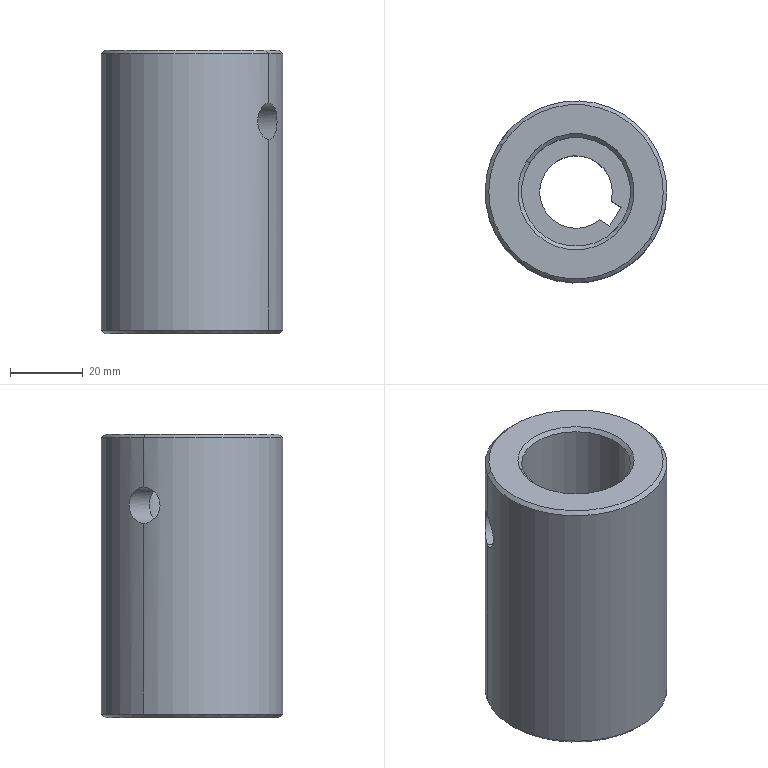Component | SolidWorks | 24-1 | 1 solid | 24 faces | box 50 x 50 x 78 mm | volume 107825 mm3 | cylinder 10 | cone 8 | plane 6 | commonest cylinder face diameters 10 x4 30 x2 20 x2 50 x2
build123d program:
from build123d import *

# Parameters (mm, degrees)
SKETCH1_R            = 25
BOSS_EXTRUDE1_DEPTH  = 78
CUT_EXTRUDE1_DEPTH   = 31
SKETCH3_R            = 15
CUT_EXTRUDE2_DEPTH   = 47
CUT_SWEEP1_PROFILE_R = 5
CHAMFER1_SIZE        = 1
CHAMFER2_SIZE        = 1
CHAMFER3_SIZE        = 1


with BuildPart() as part:
    # Sketch1 → Boss-Extrude1 (new body)
    with BuildSketch(Plane(origin=(0, 0, 0), x_dir=(1, 0, 0), z_dir=(0, 1, 0))):
        with Locations(Location((0, 0, 0), (0, 0, 270))):
            Circle(SKETCH1_R)
    extrude(amount=BOSS_EXTRUDE1_DEPTH)

    # Sketch2 → Cut-Extrude1 (cut)
    with BuildSketch(Plane(origin=(0, 78, 0), x_dir=(1, 0, 0), z_dir=(0, 1, 0))):
        with BuildLine():
            Line((3, 12.8), (-3, 12.8))
            Line((-3, 12.8), (-3, 9.539))
            ThreePointArc((-3, 9.539), (0, -10), (3, 9.539))
            Line((3, 9.539), (3, 12.8))
        make_face()
    extrude(amount=-CUT_EXTRUDE1_DEPTH, mode=Mode.SUBTRACT)

    # Sketch3 → Cut-Extrude2 (cut)
    with BuildSketch(Plane(origin=(0, 47, 0), x_dir=(1, 0, 0), z_dir=(0, 1, 0))):
        with Locations(Location((0, 0, 0), (0, 0, 270))):
            Circle(SKETCH3_R)
    extrude(amount=-CUT_EXTRUDE2_DEPTH, mode=Mode.SUBTRACT)

    # Cut-Sweep1: sweep along a path in Sketch4
    with BuildLine(Plane(origin=(0, 0, 0), x_dir=(0, 0, -1), z_dir=(1, 0, 0))) as cut_sweep1_path:
        Line((45.424, 19.5), (-33.131, 19.5))
    # Cut-Sweep1 profile (on start of the path) → Cut-Sweep1 (sweep, cut)
    with BuildSketch(Plane(origin=(0, 19.5, -45.424), x_dir=(0, 1, 0), z_dir=(0, 0, 1))):
        Circle(CUT_SWEEP1_PROFILE_R)
    sweep(path=cut_sweep1_path.line, mode=Mode.SUBTRACT)

    # Chamfer1
    chamfer1_edges = [part.edges().sort_by_distance(p)[0] for p in [
        (0, 0, -25),
        (0, 78, -25),
    ]]
    chamfer(chamfer1_edges, length=CHAMFER1_SIZE)

    # Chamfer2
    chamfer2_edges = [part.edges().sort_by_distance(p)[0] for p in [
        (0, 78, 10),
    ]]
    chamfer(chamfer2_edges, length=CHAMFER2_SIZE)

    # Chamfer3
    chamfer3_edges = [part.edges().sort_by_distance(p)[0] for p in [
        (0, 0, -15),
    ]]
    chamfer(chamfer3_edges, length=CHAMFER3_SIZE)


solid = part.part

# Placed as in the assembly
solid = solid.moved(Location((70, -47, -138.44), (-90, -57.874, 0.0002282)))